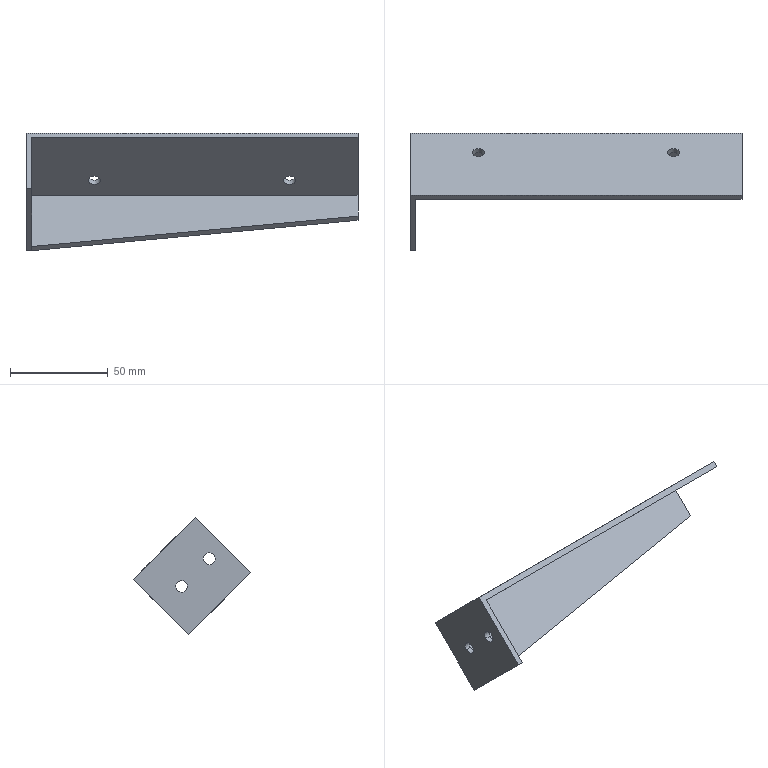Component | SolidWorks | FixedFrame-1 | 1 solid | 18 faces | box 170 x 60.1 x 60.1 mm | volume 40632 mm3 | plane 10 | cylinder 8 | commonest cylinder face diameters 6 x8
build123d program:
from build123d import *

# Parameters (mm, degrees)
SKETCH3_W           = 45
SKETCH3_H           = 3
EXTRUDE_THIN1_DEPTH = 170
SKETCH4_W           = 45
SKETCH4_H           = 40
BOSS_EXTRUDE1_DEPTH = 3
BOSS_EXTRUDE2_DEPTH = 3
SKETCH6_R           = 3
CUT_EXTRUDE1_DEPTH  = 3
SKETCH8_R           = 3
CUT_EXTRUDE2_DEPTH  = 3


with BuildPart() as part:
    # Sketch3 → Extrude-Thin1 (new body)
    with BuildSketch(Plane.XY):
        with Locations((-16.55, 24.393)):
            Rectangle(SKETCH3_W, SKETCH3_H)
    extrude(amount=EXTRUDE_THIN1_DEPTH)

    # Sketch4 → Boss-Extrude1 (add)
    with BuildSketch(Plane(origin=(0, 0, 0), x_dir=(-1, 0, 0), z_dir=(0, 0, -1))):
        with Locations((16.55, 5.893)):
            Rectangle(SKETCH4_W, SKETCH4_H)
    extrude(amount=-BOSS_EXTRUDE1_DEPTH)

    # Sketch5 → Boss-Extrude2 (add)
    with BuildSketch(Plane(origin=(5.95, 0, 0), x_dir=(0, 0, -1), z_dir=(1, 0, 0))):
        Polygon((-170, 7.893), (-3, -14.107), (-3, 22.893), (-170, 22.893), align=None)
    extrude(amount=-BOSS_EXTRUDE2_DEPTH)

    # Sketch6 → Cut-Extrude1 (cut)
    with BuildSketch(Plane.XY.offset(3)):
        with Locations((-29.05, 5.893)):
            Circle(SKETCH6_R)
        with Locations((-9.05, 5.893)):
            Circle(SKETCH6_R)
    extrude(amount=-CUT_EXTRUDE1_DEPTH, mode=Mode.SUBTRACT)

    # Sketch8 → Cut-Extrude2 (cut)
    with BuildSketch(Plane(origin=(0, 25.893, 0), x_dir=(1, 0, 0), z_dir=(0, 1, 0))):
        with Locations(Location((-8.05, -35, 0), (0, 0, 270))):
            Circle(SKETCH8_R)
        with Locations(Location((-8.05, -135, 0), (0, 0, 270))):
            Circle(SKETCH8_R)
    extrude(amount=-CUT_EXTRUDE2_DEPTH, mode=Mode.SUBTRACT)


solid = part.part

# Placed as in the assembly
solid = solid.moved(Location((490.45, -202.656, -272.987), (45, 90, 0)))
STEP:
#1=COLOUR_RGB('',0.7922,0.8196,0.9333);
#2=FILL_AREA_STYLE_COLOUR('',#1);
#3=FILL_AREA_STYLE('',(#2));
#4=SURFACE_STYLE_FILL_AREA(#3);
#5=SURFACE_SIDE_STYLE('',(#4));
#6=SURFACE_STYLE_USAGE(.BOTH.,#5);
#7=PRESENTATION_STYLE_ASSIGNMENT((#6));
#8=CARTESIAN_POINT('',(24.506,-7.565,-9.886));
#9=VERTEX_POINT('',#8);
#10=CARTESIAN_POINT('',(24.742,-7.565,-9.886));
#11=VERTEX_POINT('',#10);
#12=CARTESIAN_POINT('',(24.624,-7.565,-9.886));
#13=DIRECTION('',(0.,0.7071,0.7071));
#14=DIRECTION('',(1.,0.,0.));
#15=AXIS2_PLACEMENT_3D('',#12,#13,#14);
#16=CIRCLE('',#15,0.1181);
#17=EDGE_CURVE('',#9,#11,#16,.T.);
#18=ORIENTED_EDGE('',*,*,#17,.F.);
#19=CARTESIAN_POINT('',(24.506,-7.482,-9.803));
#20=VERTEX_POINT('',#19);
#21=CARTESIAN_POINT('',(24.506,-7.565,-9.886));
#22=DIRECTION('',(0.,0.7071,0.7071));
#23=VECTOR('',#22,39.37);
#24=LINE('',#21,#23);
#25=EDGE_CURVE('',#9,#20,#24,.T.);
#26=ORIENTED_EDGE('',*,*,#25,.T.);
#27=CARTESIAN_POINT('',(24.742,-7.482,-9.803));
#28=VERTEX_POINT('',#27);
#29=CARTESIAN_POINT('',(24.624,-7.482,-9.803));
#30=DIRECTION('',(0.,0.7071,0.7071));
#31=DIRECTION('',(1.,0.,0.));
#32=AXIS2_PLACEMENT_3D('',#29,#30,#31);
#33=CIRCLE('',#32,0.1181);
#34=EDGE_CURVE('',#20,#28,#33,.T.);
#35=ORIENTED_EDGE('',*,*,#34,.T.);
#36=CARTESIAN_POINT('',(24.742,-7.565,-9.886));
#37=DIRECTION('',(0.,0.7071,0.7071));
#38=VECTOR('',#37,39.37);
#39=LINE('',#36,#38);
#40=EDGE_CURVE('',#11,#28,#39,.T.);
#41=ORIENTED_EDGE('',*,*,#40,.F.);
#42=EDGE_LOOP('',(#18,#26,#35,#41));
#43=FACE_OUTER_BOUND('',#42,.T.);
#44=CARTESIAN_POINT('',(24.624,-7.565,-9.886));
#45=DIRECTION('',(0.,0.7071,0.7071));
#46=DIRECTION('',(1.,0.,0.));
#47=AXIS2_PLACEMENT_3D('',#44,#45,#46);
#48=CYLINDRICAL_SURFACE('',#47,0.1181);
#49=ADVANCED_FACE('',(#43),#48,.F.);
#50=CARTESIAN_POINT('',(20.569,-7.565,-9.886));
#51=VERTEX_POINT('',#50);
#52=CARTESIAN_POINT('',(20.805,-7.565,-9.886));
#53=VERTEX_POINT('',#52);
#54=CARTESIAN_POINT('',(20.687,-7.565,-9.886));
#55=DIRECTION('',(0.,0.7071,0.7071));
#56=DIRECTION('',(1.,0.,0.));
#57=AXIS2_PLACEMENT_3D('',#54,#55,#56);
#58=CIRCLE('',#57,0.1181);
#59=EDGE_CURVE('',#51,#53,#58,.T.);
#60=ORIENTED_EDGE('',*,*,#59,.F.);
#61=CARTESIAN_POINT('',(20.569,-7.482,-9.803));
#62=VERTEX_POINT('',#61);
#63=CARTESIAN_POINT('',(20.569,-7.565,-9.886));
#64=DIRECTION('',(0.,0.7071,0.7071));
#65=VECTOR('',#64,39.37);
#66=LINE('',#63,#65);
#67=EDGE_CURVE('',#51,#62,#66,.T.);
#68=ORIENTED_EDGE('',*,*,#67,.T.);
#69=CARTESIAN_POINT('',(20.805,-7.482,-9.803));
#70=VERTEX_POINT('',#69);
#71=CARTESIAN_POINT('',(20.687,-7.482,-9.803));
#72=DIRECTION('',(0.,0.7071,0.7071));
#73=DIRECTION('',(1.,0.,0.));
#74=AXIS2_PLACEMENT_3D('',#71,#72,#73);
#75=CIRCLE('',#74,0.1181);
#76=EDGE_CURVE('',#62,#70,#75,.T.);
#77=ORIENTED_EDGE('',*,*,#76,.T.);
#78=CARTESIAN_POINT('',(20.805,-7.565,-9.886));
#79=DIRECTION('',(0.,0.7071,0.7071));
#80=VECTOR('',#79,39.37);
#81=LINE('',#78,#80);
#82=EDGE_CURVE('',#53,#70,#81,.T.);
#83=ORIENTED_EDGE('',*,*,#82,.F.);
#84=EDGE_LOOP('',(#60,#68,#77,#83));
#85=FACE_OUTER_BOUND('',#84,.T.);
#86=CARTESIAN_POINT('',(20.687,-7.565,-9.886));
#87=DIRECTION('',(0.,0.7071,0.7071));
#88=DIRECTION('',(1.,0.,0.));
#89=AXIS2_PLACEMENT_3D('',#86,#87,#88);
#90=CYLINDRICAL_SURFACE('',#89,0.1181);
#91=ADVANCED_FACE('',(#85),#90,.F.);
#92=CARTESIAN_POINT('',(19.309,-8.15,-10.248));
#93=VERTEX_POINT('',#92);
#94=CARTESIAN_POINT('',(19.309,-7.983,-10.415));
#95=VERTEX_POINT('',#94);
#96=CARTESIAN_POINT('',(19.309,-8.066,-10.332));
#97=DIRECTION('',(1.,-0.,-0.));
#98=DIRECTION('',(0.,0.7071,-0.7071));
#99=AXIS2_PLACEMENT_3D('',#96,#97,#98);
#100=CIRCLE('',#99,0.1181);
#101=EDGE_CURVE('',#93,#95,#100,.T.);
#102=ORIENTED_EDGE('',*,*,#101,.F.);
#103=CARTESIAN_POINT('',(19.427,-8.15,-10.248));
#104=VERTEX_POINT('',#103);
#105=CARTESIAN_POINT('',(19.309,-8.15,-10.248));
#106=DIRECTION('',(1.,-0.,-0.));
#107=VECTOR('',#106,39.37);
#108=LINE('',#105,#107);
#109=EDGE_CURVE('',#93,#104,#108,.T.);
#110=ORIENTED_EDGE('',*,*,#109,.T.);
#111=CARTESIAN_POINT('',(19.427,-7.983,-10.415));
#112=VERTEX_POINT('',#111);
#113=CARTESIAN_POINT('',(19.427,-8.066,-10.332));
#114=DIRECTION('',(1.,-0.,-0.));
#115=DIRECTION('',(0.,0.7071,-0.7071));
#116=AXIS2_PLACEMENT_3D('',#113,#114,#115);
#117=CIRCLE('',#116,0.1181);
#118=EDGE_CURVE('',#104,#112,#117,.T.);
#119=ORIENTED_EDGE('',*,*,#118,.T.);
#120=CARTESIAN_POINT('',(19.309,-7.983,-10.415));
#121=DIRECTION('',(1.,-0.,-0.));
#122=VECTOR('',#121,39.37);
#123=LINE('',#120,#122);
#124=EDGE_CURVE('',#95,#112,#123,.T.);
#125=ORIENTED_EDGE('',*,*,#124,.F.);
#126=EDGE_LOOP('',(#102,#110,#119,#125));
#127=FACE_OUTER_BOUND('',#126,.T.);
#128=CARTESIAN_POINT('',(19.309,-8.066,-10.332));
#129=DIRECTION('',(1.,-0.,-0.));
#130=DIRECTION('',(0.,0.7071,-0.7071));
#131=AXIS2_PLACEMENT_3D('',#128,#129,#130);
#132=CYLINDRICAL_SURFACE('',#131,0.1181);
#133=ADVANCED_FACE('',(#127),#132,.F.);
#134=CARTESIAN_POINT('',(19.309,-8.707,-9.691));
#135=VERTEX_POINT('',#134);
#136=CARTESIAN_POINT('',(19.309,-8.54,-9.858));
#137=VERTEX_POINT('',#136);
#138=CARTESIAN_POINT('',(19.309,-8.623,-9.775));
#139=DIRECTION('',(1.,-0.,-0.));
#140=DIRECTION('',(0.,0.7071,-0.7071));
#141=AXIS2_PLACEMENT_3D('',#138,#139,#140);
#142=CIRCLE('',#141,0.1181);
#143=EDGE_CURVE('',#135,#137,#142,.T.);
#144=ORIENTED_EDGE('',*,*,#143,.F.);
#145=CARTESIAN_POINT('',(19.427,-8.707,-9.691));
#146=VERTEX_POINT('',#145);
#147=CARTESIAN_POINT('',(19.309,-8.707,-9.691));
#148=DIRECTION('',(1.,-0.,-0.));
#149=VECTOR('',#148,39.37);
#150=LINE('',#147,#149);
#151=EDGE_CURVE('',#135,#146,#150,.T.);
#152=ORIENTED_EDGE('',*,*,#151,.T.);
#153=CARTESIAN_POINT('',(19.427,-8.54,-9.858));
#154=VERTEX_POINT('',#153);
#155=CARTESIAN_POINT('',(19.427,-8.623,-9.775));
#156=DIRECTION('',(1.,-0.,-0.));
#157=DIRECTION('',(0.,0.7071,-0.7071));
#158=AXIS2_PLACEMENT_3D('',#155,#156,#157);
#159=CIRCLE('',#158,0.1181);
#160=EDGE_CURVE('',#146,#154,#159,.T.);
#161=ORIENTED_EDGE('',*,*,#160,.T.);
#162=CARTESIAN_POINT('',(19.309,-8.54,-9.858));
#163=DIRECTION('',(1.,-0.,-0.));
#164=VECTOR('',#163,39.37);
#165=LINE('',#162,#164);
#166=EDGE_CURVE('',#137,#154,#165,.T.);
#167=ORIENTED_EDGE('',*,*,#166,.F.);
#168=EDGE_LOOP('',(#144,#152,#161,#167));
#169=FACE_OUTER_BOUND('',#168,.T.);
#170=CARTESIAN_POINT('',(19.309,-8.623,-9.775));
#171=DIRECTION('',(1.,-0.,-0.));
#172=DIRECTION('',(0.,0.7071,-0.7071));
#173=AXIS2_PLACEMENT_3D('',#170,#171,#172);
#174=CYLINDRICAL_SURFACE('',#173,0.1181);
#175=ADVANCED_FACE('',(#169),#174,.F.);
#176=CARTESIAN_POINT('',(24.624,-7.565,-9.886));
#177=DIRECTION('',(0.,0.7071,0.7071));
#178=DIRECTION('',(1.,0.,0.));
#179=AXIS2_PLACEMENT_3D('',#176,#177,#178);
#180=CIRCLE('',#179,0.1181);
#181=EDGE_CURVE('',#11,#9,#180,.T.);
#182=ORIENTED_EDGE('',*,*,#181,.T.);
#183=ORIENTED_EDGE('',*,*,#17,.T.);
#184=EDGE_LOOP('',(#182,#183));
#185=FACE_BOUND('',#184,.T.);
#186=CARTESIAN_POINT('',(20.687,-7.565,-9.886));
#187=DIRECTION('',(0.,0.7071,0.7071));
#188=DIRECTION('',(1.,0.,0.));
#189=AXIS2_PLACEMENT_3D('',#186,#187,#188);
#190=CIRCLE('',#189,0.1181);
#191=EDGE_CURVE('',#53,#51,#190,.T.);
#192=ORIENTED_EDGE('',*,*,#191,.T.);
#193=ORIENTED_EDGE('',*,*,#59,.T.);
#194=EDGE_LOOP('',(#192,#193));
#195=FACE_BOUND('',#194,.T.);
#196=CARTESIAN_POINT('',(19.427,-7.259,-10.192));
#197=VERTEX_POINT('',#196);
#198=CARTESIAN_POINT('',(26.002,-7.259,-10.192));
#199=VERTEX_POINT('',#198);
#200=CARTESIAN_POINT('',(19.427,-7.259,-10.192));
#201=DIRECTION('',(1.,-0.,-0.));
#202=VECTOR('',#201,39.37);
#203=LINE('',#200,#202);
#204=EDGE_CURVE('',#197,#199,#203,.T.);
#205=ORIENTED_EDGE('',*,*,#204,.T.);
#206=CARTESIAN_POINT('',(26.002,-8.428,-9.023));
#207=VERTEX_POINT('',#206);
#208=CARTESIAN_POINT('',(26.002,-8.428,-9.023));
#209=DIRECTION('',(-0.,0.7071,-0.7071));
#210=VECTOR('',#209,39.37);
#211=LINE('',#208,#210);
#212=EDGE_CURVE('',#207,#199,#211,.T.);
#213=ORIENTED_EDGE('',*,*,#212,.F.);
#214=CARTESIAN_POINT('',(19.427,-8.428,-9.023));
#215=VERTEX_POINT('',#214);
#216=CARTESIAN_POINT('',(26.002,-8.428,-9.023));
#217=DIRECTION('',(-1.,0.,0.));
#218=VECTOR('',#217,39.37);
#219=LINE('',#216,#218);
#220=EDGE_CURVE('',#207,#215,#219,.T.);
#221=ORIENTED_EDGE('',*,*,#220,.T.);
#222=CARTESIAN_POINT('',(19.427,-8.428,-9.023));
#223=DIRECTION('',(0.,-0.7071,0.7071));
#224=VECTOR('',#223,39.37);
#225=LINE('',#222,#224);
#226=EDGE_CURVE('',#197,#215,#225,.T.);
#227=ORIENTED_EDGE('',*,*,#226,.F.);
#228=EDGE_LOOP('',(#205,#213,#221,#227));
#229=FACE_OUTER_BOUND('',#228,.T.);
#230=CARTESIAN_POINT('',(26.002,-8.428,-9.023));
#231=DIRECTION('',(0.,0.7071,0.7071));
#232=DIRECTION('',(1.,-0.,-0.));
#233=AXIS2_PLACEMENT_3D('',#230,#231,#232);
#234=PLANE('',#233);
#235=ADVANCED_FACE('',(#185,#195,#229),#234,.F.);
#236=CARTESIAN_POINT('',(19.427,-8.066,-10.332));
#237=DIRECTION('',(1.,-0.,-0.));
#238=DIRECTION('',(0.,0.7071,-0.7071));
#239=AXIS2_PLACEMENT_3D('',#236,#237,#238);
#240=CIRCLE('',#239,0.1181);
#241=EDGE_CURVE('',#112,#104,#240,.T.);
#242=ORIENTED_EDGE('',*,*,#241,.F.);
#243=ORIENTED_EDGE('',*,*,#118,.F.);
#244=EDGE_LOOP('',(#242,#243));
#245=FACE_BOUND('',#244,.T.);
#246=CARTESIAN_POINT('',(19.427,-8.623,-9.775));
#247=DIRECTION('',(1.,-0.,-0.));
#248=DIRECTION('',(0.,0.7071,-0.7071));
#249=AXIS2_PLACEMENT_3D('',#246,#247,#248);
#250=CIRCLE('',#249,0.1181);
#251=EDGE_CURVE('',#154,#146,#250,.T.);
#252=ORIENTED_EDGE('',*,*,#251,.F.);
#253=ORIENTED_EDGE('',*,*,#160,.F.);
#254=EDGE_LOOP('',(#252,#253));
#255=FACE_BOUND('',#254,.T.);
#256=CARTESIAN_POINT('',(19.427,-8.289,-11.222));
#257=VERTEX_POINT('',#256);
#258=CARTESIAN_POINT('',(19.427,-8.289,-11.222));
#259=DIRECTION('',(0.,0.7071,0.7071));
#260=VECTOR('',#259,39.37);
#261=LINE('',#258,#260);
#262=EDGE_CURVE('',#257,#197,#261,.T.);
#263=ORIENTED_EDGE('',*,*,#262,.T.);
#264=ORIENTED_EDGE('',*,*,#226,.T.);
#265=CARTESIAN_POINT('',(19.427,-9.458,-10.053));
#266=VERTEX_POINT('',#265);
#267=CARTESIAN_POINT('',(19.427,-8.345,-8.94));
#268=DIRECTION('',(0.,0.7071,0.7071));
#269=VECTOR('',#268,39.37);
#270=LINE('',#267,#269);
#271=EDGE_CURVE('',#266,#215,#270,.T.);
#272=ORIENTED_EDGE('',*,*,#271,.F.);
#273=CARTESIAN_POINT('',(19.427,-8.206,-11.306));
#274=DIRECTION('',(0.,-0.7071,0.7071));
#275=VECTOR('',#274,39.37);
#276=LINE('',#273,#275);
#277=EDGE_CURVE('',#257,#266,#276,.T.);
#278=ORIENTED_EDGE('',*,*,#277,.F.);
#279=EDGE_LOOP('',(#263,#264,#272,#278));
#280=FACE_OUTER_BOUND('',#279,.T.);
#281=CARTESIAN_POINT('',(19.427,-7.979,-10.748));
#282=DIRECTION('',(-1.,0.,0.));
#283=DIRECTION('',(0.,-0.7071,0.7071));
#284=AXIS2_PLACEMENT_3D('',#281,#282,#283);
#285=PLANE('',#284);
#286=ADVANCED_FACE('',(#245,#255,#280),#285,.F.);
#287=CARTESIAN_POINT('',(19.309,-7.092,-10.192));
#288=VERTEX_POINT('',#287);
#289=CARTESIAN_POINT('',(19.309,-8.206,-11.306));
#290=VERTEX_POINT('',#289);
#291=CARTESIAN_POINT('',(19.309,-7.092,-10.192));
#292=DIRECTION('',(-0.,-0.7071,-0.7071));
#293=VECTOR('',#292,39.37);
#294=LINE('',#291,#293);
#295=EDGE_CURVE('',#288,#290,#294,.T.);
#296=ORIENTED_EDGE('',*,*,#295,.F.);
#297=CARTESIAN_POINT('',(26.002,-7.092,-10.192));
#298=VERTEX_POINT('',#297);
#299=CARTESIAN_POINT('',(26.002,-7.092,-10.192));
#300=DIRECTION('',(-1.,0.,0.));
#301=VECTOR('',#300,39.37);
#302=LINE('',#299,#301);
#303=EDGE_CURVE('',#298,#288,#302,.T.);
#304=ORIENTED_EDGE('',*,*,#303,.F.);
#305=CARTESIAN_POINT('',(26.002,-7.593,-10.693));
#306=VERTEX_POINT('',#305);
#307=CARTESIAN_POINT('',(26.002,-7.092,-10.192));
#308=DIRECTION('',(-0.,-0.7071,-0.7071));
#309=VECTOR('',#308,39.37);
#310=LINE('',#307,#309);
#311=EDGE_CURVE('',#298,#306,#310,.T.);
#312=ORIENTED_EDGE('',*,*,#311,.T.);
#313=CARTESIAN_POINT('',(19.427,-8.206,-11.306));
#314=VERTEX_POINT('',#313);
#315=CARTESIAN_POINT('',(26.002,-7.593,-10.693));
#316=DIRECTION('',(-0.9914,-0.09235,-0.09235));
#317=VECTOR('',#316,39.37);
#318=LINE('',#315,#317);
#319=EDGE_CURVE('',#306,#314,#318,.T.);
#320=ORIENTED_EDGE('',*,*,#319,.T.);
#321=CARTESIAN_POINT('',(19.427,-8.206,-11.306));
#322=DIRECTION('',(-1.,0.,0.));
#323=VECTOR('',#322,39.37);
#324=LINE('',#321,#323);
#325=EDGE_CURVE('',#314,#290,#324,.T.);
#326=ORIENTED_EDGE('',*,*,#325,.T.);
#327=EDGE_LOOP('',(#296,#304,#312,#320,#326));
#328=FACE_OUTER_BOUND('',#327,.T.);
#329=CARTESIAN_POINT('',(26.002,-7.092,-10.192));
#330=DIRECTION('',(0.,0.7071,-0.7071));
#331=DIRECTION('',(-1.,0.,0.));
#332=AXIS2_PLACEMENT_3D('',#329,#330,#331);
#333=PLANE('',#332);
#334=ADVANCED_FACE('',(#328),#333,.T.);
#335=CARTESIAN_POINT('',(24.624,-7.482,-9.803));
#336=DIRECTION('',(0.,0.7071,0.7071));
#337=DIRECTION('',(1.,0.,0.));
#338=AXIS2_PLACEMENT_3D('',#335,#336,#337);
#339=CIRCLE('',#338,0.1181);
#340=EDGE_CURVE('',#28,#20,#339,.T.);
#341=ORIENTED_EDGE('',*,*,#340,.F.);
#342=ORIENTED_EDGE('',*,*,#34,.F.);
#343=EDGE_LOOP('',(#341,#342));
#344=FACE_BOUND('',#343,.T.);
#345=CARTESIAN_POINT('',(20.687,-7.482,-9.803));
#346=DIRECTION('',(0.,0.7071,0.7071));
#347=DIRECTION('',(1.,0.,0.));
#348=AXIS2_PLACEMENT_3D('',#345,#346,#347);
#349=CIRCLE('',#348,0.1181);
#350=EDGE_CURVE('',#70,#62,#349,.T.);
#351=ORIENTED_EDGE('',*,*,#350,.F.);
#352=ORIENTED_EDGE('',*,*,#76,.F.);
#353=EDGE_LOOP('',(#351,#352));
#354=FACE_BOUND('',#353,.T.);
#355=CARTESIAN_POINT('',(19.309,-8.345,-8.94));
#356=VERTEX_POINT('',#355);
#357=CARTESIAN_POINT('',(19.309,-8.345,-8.94));
#358=DIRECTION('',(-0.,0.7071,-0.7071));
#359=VECTOR('',#358,39.37);
#360=LINE('',#357,#359);
#361=EDGE_CURVE('',#356,#288,#360,.T.);
#362=ORIENTED_EDGE('',*,*,#361,.F.);
#363=CARTESIAN_POINT('',(26.002,-8.345,-8.94));
#364=VERTEX_POINT('',#363);
#365=CARTESIAN_POINT('',(26.002,-8.345,-8.94));
#366=DIRECTION('',(-1.,0.,0.));
#367=VECTOR('',#366,39.37);
#368=LINE('',#365,#367);
#369=EDGE_CURVE('',#364,#356,#368,.T.);
#370=ORIENTED_EDGE('',*,*,#369,.F.);
#371=CARTESIAN_POINT('',(26.002,-8.345,-8.94));
#372=DIRECTION('',(-0.,0.7071,-0.7071));
#373=VECTOR('',#372,39.37);
#374=LINE('',#371,#373);
#375=EDGE_CURVE('',#364,#298,#374,.T.);
#376=ORIENTED_EDGE('',*,*,#375,.T.);
#377=ORIENTED_EDGE('',*,*,#303,.T.);
#378=EDGE_LOOP('',(#362,#370,#376,#377));
#379=FACE_OUTER_BOUND('',#378,.T.);
#380=CARTESIAN_POINT('',(26.002,-8.345,-8.94));
#381=DIRECTION('',(0.,0.7071,0.7071));
#382=DIRECTION('',(1.,-0.,-0.));
#383=AXIS2_PLACEMENT_3D('',#380,#381,#382);
#384=PLANE('',#383);
#385=ADVANCED_FACE('',(#344,#354,#379),#384,.T.);
#386=CARTESIAN_POINT('',(19.309,-9.458,-10.053));
#387=VERTEX_POINT('',#386);
#388=CARTESIAN_POINT('',(19.309,-8.428,-9.023));
#389=DIRECTION('',(0.,0.7071,0.7071));
#390=VECTOR('',#389,39.37);
#391=LINE('',#388,#390);
#392=EDGE_CURVE('',#387,#356,#391,.T.);
#393=ORIENTED_EDGE('',*,*,#392,.F.);
#394=CARTESIAN_POINT('',(19.427,-9.458,-10.053));
#395=DIRECTION('',(-1.,0.,0.));
#396=VECTOR('',#395,39.37);
#397=LINE('',#394,#396);
#398=EDGE_CURVE('',#266,#387,#397,.T.);
#399=ORIENTED_EDGE('',*,*,#398,.F.);
#400=ORIENTED_EDGE('',*,*,#271,.T.);
#401=ORIENTED_EDGE('',*,*,#220,.F.);
#402=CARTESIAN_POINT('',(26.002,-8.428,-9.023));
#403=DIRECTION('',(0.,0.7071,0.7071));
#404=VECTOR('',#403,39.37);
#405=LINE('',#402,#404);
#406=EDGE_CURVE('',#207,#364,#405,.T.);
#407=ORIENTED_EDGE('',*,*,#406,.T.);
#408=ORIENTED_EDGE('',*,*,#369,.T.);
#409=EDGE_LOOP('',(#393,#399,#400,#401,#407,#408));
#410=FACE_OUTER_BOUND('',#409,.T.);
#411=CARTESIAN_POINT('',(26.002,-8.428,-9.023));
#412=DIRECTION('',(-0.,-0.7071,0.7071));
#413=DIRECTION('',(1.,-0.,-0.));
#414=AXIS2_PLACEMENT_3D('',#411,#412,#413);
#415=PLANE('',#414);
#416=ADVANCED_FACE('',(#410),#415,.T.);
#417=ORIENTED_EDGE('',*,*,#212,.T.);
#418=CARTESIAN_POINT('',(26.002,-7.677,-10.61));
#419=VERTEX_POINT('',#418);
#420=CARTESIAN_POINT('',(26.002,-7.259,-10.192));
#421=DIRECTION('',(-0.,-0.7071,-0.7071));
#422=VECTOR('',#421,39.37);
#423=LINE('',#420,#422);
#424=EDGE_CURVE('',#199,#419,#423,.T.);
#425=ORIENTED_EDGE('',*,*,#424,.T.);
#426=CARTESIAN_POINT('',(26.002,-7.677,-10.61));
#427=DIRECTION('',(-0.,0.7071,-0.7071));
#428=VECTOR('',#427,39.37);
#429=LINE('',#426,#428);
#430=EDGE_CURVE('',#419,#306,#429,.T.);
#431=ORIENTED_EDGE('',*,*,#430,.T.);
#432=ORIENTED_EDGE('',*,*,#311,.F.);
#433=ORIENTED_EDGE('',*,*,#375,.F.);
#434=ORIENTED_EDGE('',*,*,#406,.F.);
#435=EDGE_LOOP('',(#417,#425,#431,#432,#433,#434));
#436=FACE_OUTER_BOUND('',#435,.T.);
#437=CARTESIAN_POINT('',(26.002,-7.979,-10.748));
#438=DIRECTION('',(-1.,0.,0.));
#439=DIRECTION('',(0.,-0.7071,0.7071));
#440=AXIS2_PLACEMENT_3D('',#437,#438,#439);
#441=PLANE('',#440);
#442=ADVANCED_FACE('',(#436),#441,.F.);
#443=CARTESIAN_POINT('',(19.309,-8.066,-10.332));
#444=DIRECTION('',(1.,-0.,-0.));
#445=DIRECTION('',(0.,0.7071,-0.7071));
#446=AXIS2_PLACEMENT_3D('',#443,#444,#445);
#447=CIRCLE('',#446,0.1181);
#448=EDGE_CURVE('',#95,#93,#447,.T.);
#449=ORIENTED_EDGE('',*,*,#448,.T.);
#450=ORIENTED_EDGE('',*,*,#101,.T.);
#451=EDGE_LOOP('',(#449,#450));
#452=FACE_BOUND('',#451,.T.);
#453=CARTESIAN_POINT('',(19.309,-8.623,-9.775));
#454=DIRECTION('',(1.,-0.,-0.));
#455=DIRECTION('',(0.,0.7071,-0.7071));
#456=AXIS2_PLACEMENT_3D('',#453,#454,#455);
#457=CIRCLE('',#456,0.1181);
#458=EDGE_CURVE('',#137,#135,#457,.T.);
#459=ORIENTED_EDGE('',*,*,#458,.T.);
#460=ORIENTED_EDGE('',*,*,#143,.T.);
#461=EDGE_LOOP('',(#459,#460));
#462=FACE_BOUND('',#461,.T.);
#463=ORIENTED_EDGE('',*,*,#295,.T.);
#464=CARTESIAN_POINT('',(19.309,-8.206,-11.306));
#465=DIRECTION('',(0.,-0.7071,0.7071));
#466=VECTOR('',#465,39.37);
#467=LINE('',#464,#466);
#468=EDGE_CURVE('',#290,#387,#467,.T.);
#469=ORIENTED_EDGE('',*,*,#468,.T.);
#470=ORIENTED_EDGE('',*,*,#392,.T.);
#471=ORIENTED_EDGE('',*,*,#361,.T.);
#472=EDGE_LOOP('',(#463,#469,#470,#471));
#473=FACE_OUTER_BOUND('',#472,.T.);
#474=CARTESIAN_POINT('',(19.309,-7.979,-10.748));
#475=DIRECTION('',(-1.,0.,0.));
#476=DIRECTION('',(0.,-0.7071,0.7071));
#477=AXIS2_PLACEMENT_3D('',#474,#475,#476);
#478=PLANE('',#477);
#479=ADVANCED_FACE('',(#452,#462,#473),#478,.T.);
#480=ORIENTED_EDGE('',*,*,#468,.F.);
#481=ORIENTED_EDGE('',*,*,#325,.F.);
#482=CARTESIAN_POINT('',(19.427,-8.206,-11.306));
#483=DIRECTION('',(0.,-0.7071,0.7071));
#484=VECTOR('',#483,39.37);
#485=LINE('',#482,#484);
#486=EDGE_CURVE('',#314,#257,#485,.T.);
#487=ORIENTED_EDGE('',*,*,#486,.T.);
#488=ORIENTED_EDGE('',*,*,#277,.T.);
#489=ORIENTED_EDGE('',*,*,#398,.T.);
#490=EDGE_LOOP('',(#480,#481,#487,#488,#489));
#491=FACE_OUTER_BOUND('',#490,.T.);
#492=CARTESIAN_POINT('',(19.427,-8.206,-11.306));
#493=DIRECTION('',(-0.,-0.7071,-0.7071));
#494=DIRECTION('',(-0.,0.7071,-0.7071));
#495=AXIS2_PLACEMENT_3D('',#492,#493,#494);
#496=PLANE('',#495);
#497=ADVANCED_FACE('',(#491),#496,.T.);
#498=ORIENTED_EDGE('',*,*,#319,.F.);
#499=ORIENTED_EDGE('',*,*,#430,.F.);
#500=CARTESIAN_POINT('',(26.002,-7.677,-10.61));
#501=DIRECTION('',(-0.9914,-0.09235,-0.09235));
#502=VECTOR('',#501,39.37);
#503=LINE('',#500,#502);
#504=EDGE_CURVE('',#419,#257,#503,.T.);
#505=ORIENTED_EDGE('',*,*,#504,.T.);
#506=ORIENTED_EDGE('',*,*,#486,.F.);
#507=EDGE_LOOP('',(#498,#499,#505,#506));
#508=FACE_OUTER_BOUND('',#507,.T.);
#509=CARTESIAN_POINT('',(26.002,-7.677,-10.61));
#510=DIRECTION('',(0.1306,-0.701,-0.701));
#511=DIRECTION('',(-0.9914,-0.09235,-0.09235));
#512=AXIS2_PLACEMENT_3D('',#509,#510,#511);
#513=PLANE('',#512);
#514=ADVANCED_FACE('',(#508),#513,.T.);
#515=ORIENTED_EDGE('',*,*,#262,.F.);
#516=ORIENTED_EDGE('',*,*,#504,.F.);
#517=ORIENTED_EDGE('',*,*,#424,.F.);
#518=ORIENTED_EDGE('',*,*,#204,.F.);
#519=EDGE_LOOP('',(#515,#516,#517,#518));
#520=FACE_OUTER_BOUND('',#519,.T.);
#521=CARTESIAN_POINT('',(19.309,-7.896,-10.83));
#522=DIRECTION('',(0.,0.7071,-0.7071));
#523=DIRECTION('',(-1.,0.,0.));
#524=AXIS2_PLACEMENT_3D('',#521,#522,#523);
#525=PLANE('',#524);
#526=ADVANCED_FACE('',(#520),#525,.F.);
#527=ORIENTED_EDGE('',*,*,#151,.F.);
#528=ORIENTED_EDGE('',*,*,#458,.F.);
#529=ORIENTED_EDGE('',*,*,#166,.T.);
#530=ORIENTED_EDGE('',*,*,#251,.T.);
#531=EDGE_LOOP('',(#527,#528,#529,#530));
#532=FACE_OUTER_BOUND('',#531,.T.);
#533=CARTESIAN_POINT('',(19.309,-8.623,-9.775));
#534=DIRECTION('',(1.,-0.,-0.));
#535=DIRECTION('',(0.,0.7071,-0.7071));
#536=AXIS2_PLACEMENT_3D('',#533,#534,#535);
#537=CYLINDRICAL_SURFACE('',#536,0.1181);
#538=ADVANCED_FACE('',(#532),#537,.F.);
#539=ORIENTED_EDGE('',*,*,#109,.F.);
#540=ORIENTED_EDGE('',*,*,#448,.F.);
#541=ORIENTED_EDGE('',*,*,#124,.T.);
#542=ORIENTED_EDGE('',*,*,#241,.T.);
#543=EDGE_LOOP('',(#539,#540,#541,#542));
#544=FACE_OUTER_BOUND('',#543,.T.);
#545=CARTESIAN_POINT('',(19.309,-8.066,-10.332));
#546=DIRECTION('',(1.,-0.,-0.));
#547=DIRECTION('',(0.,0.7071,-0.7071));
#548=AXIS2_PLACEMENT_3D('',#545,#546,#547);
#549=CYLINDRICAL_SURFACE('',#548,0.1181);
#550=ADVANCED_FACE('',(#544),#549,.F.);
#551=ORIENTED_EDGE('',*,*,#67,.F.);
#552=ORIENTED_EDGE('',*,*,#191,.F.);
#553=ORIENTED_EDGE('',*,*,#82,.T.);
#554=ORIENTED_EDGE('',*,*,#350,.T.);
#555=EDGE_LOOP('',(#551,#552,#553,#554));
#556=FACE_OUTER_BOUND('',#555,.T.);
#557=CARTESIAN_POINT('',(20.687,-7.565,-9.886));
#558=DIRECTION('',(0.,0.7071,0.7071));
#559=DIRECTION('',(1.,0.,0.));
#560=AXIS2_PLACEMENT_3D('',#557,#558,#559);
#561=CYLINDRICAL_SURFACE('',#560,0.1181);
#562=ADVANCED_FACE('',(#556),#561,.F.);
#563=ORIENTED_EDGE('',*,*,#25,.F.);
#564=ORIENTED_EDGE('',*,*,#181,.F.);
#565=ORIENTED_EDGE('',*,*,#40,.T.);
#566=ORIENTED_EDGE('',*,*,#340,.T.);
#567=EDGE_LOOP('',(#563,#564,#565,#566));
#568=FACE_OUTER_BOUND('',#567,.T.);
#569=CARTESIAN_POINT('',(24.624,-7.565,-9.886));
#570=DIRECTION('',(0.,0.7071,0.7071));
#571=DIRECTION('',(1.,0.,0.));
#572=AXIS2_PLACEMENT_3D('',#569,#570,#571);
#573=CYLINDRICAL_SURFACE('',#572,0.1181);
#574=ADVANCED_FACE('',(#568),#573,.F.);
#575=CLOSED_SHELL('',(#49,#91,#133,#175,#235,#286,#334,#385,#416,#442,#479,#497,#514,#526,#538,#550,#562,#574));
#576=MANIFOLD_SOLID_BREP('',#575);
#577=STYLED_ITEM('',(#7),#576);
#578=(LENGTH_UNIT()NAMED_UNIT(*)SI_UNIT($,.METRE.));
#579=LENGTH_MEASURE_WITH_UNIT(LENGTH_MEASURE(0.0254),#578);
#580=DIMENSIONAL_EXPONENTS(1.,0.,0.,0.,0.,0.,0.);
#581=(CONVERSION_BASED_UNIT('',#579)LENGTH_UNIT()NAMED_UNIT(#580));
#582=UNCERTAINTY_MEASURE_WITH_UNIT(LENGTH_MEASURE(0.00001),#581,'','');
#583=(NAMED_UNIT(*)PLANE_ANGLE_UNIT()SI_UNIT($,.RADIAN.));
#584=(NAMED_UNIT(*)SI_UNIT($,.STERADIAN.)SOLID_ANGLE_UNIT());
#585=(GEOMETRIC_REPRESENTATION_CONTEXT(3)GLOBAL_UNCERTAINTY_ASSIGNED_CONTEXT((#582))GLOBAL_UNIT_ASSIGNED_CONTEXT((#581,#583,#584))REPRESENTATION_CONTEXT('',''));
#586=MECHANICAL_DESIGN_GEOMETRIC_PRESENTATION_REPRESENTATION('',(#577),#585);
#587=PRESENTATION_LAYER_ASSIGNMENT('','',(#577));
#588=CARTESIAN_POINT('',(0.,0.,0.));
#589=DIRECTION('',(0.,0.,1.));
#590=DIRECTION('',(1.,0.,0.));
#591=AXIS2_PLACEMENT_3D('',#588,#589,#590);
#592=(LENGTH_UNIT()NAMED_UNIT(*)SI_UNIT($,.METRE.));
#593=LENGTH_MEASURE_WITH_UNIT(LENGTH_MEASURE(0.0254),#592);
#594=DIMENSIONAL_EXPONENTS(1.,0.,0.,0.,0.,0.,0.);
#595=(CONVERSION_BASED_UNIT('',#593)LENGTH_UNIT()NAMED_UNIT(#594));
#596=UNCERTAINTY_MEASURE_WITH_UNIT(LENGTH_MEASURE(0.00001),#595,'','');
#597=(NAMED_UNIT(*)PLANE_ANGLE_UNIT()SI_UNIT($,.RADIAN.));
#598=(NAMED_UNIT(*)SI_UNIT($,.STERADIAN.)SOLID_ANGLE_UNIT());
#599=(GEOMETRIC_REPRESENTATION_CONTEXT(3)GLOBAL_UNCERTAINTY_ASSIGNED_CONTEXT((#596))GLOBAL_UNIT_ASSIGNED_CONTEXT((#595,#597,#598))REPRESENTATION_CONTEXT('',''));
#600=ADVANCED_BREP_SHAPE_REPRESENTATION('',(#576,#591),#599);